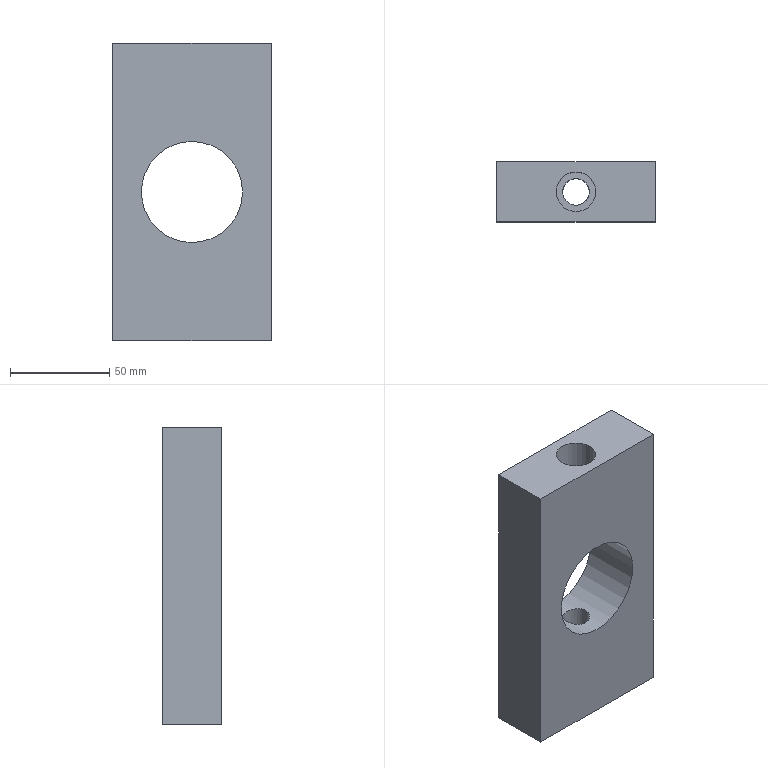Component | NX | BRACKET | 1 solid | 11 faces | volume 278868 mm3 | plane 7 | cylinder 4 | commonest cylinder face diameters 13.5 x2 51 x1 20 x1